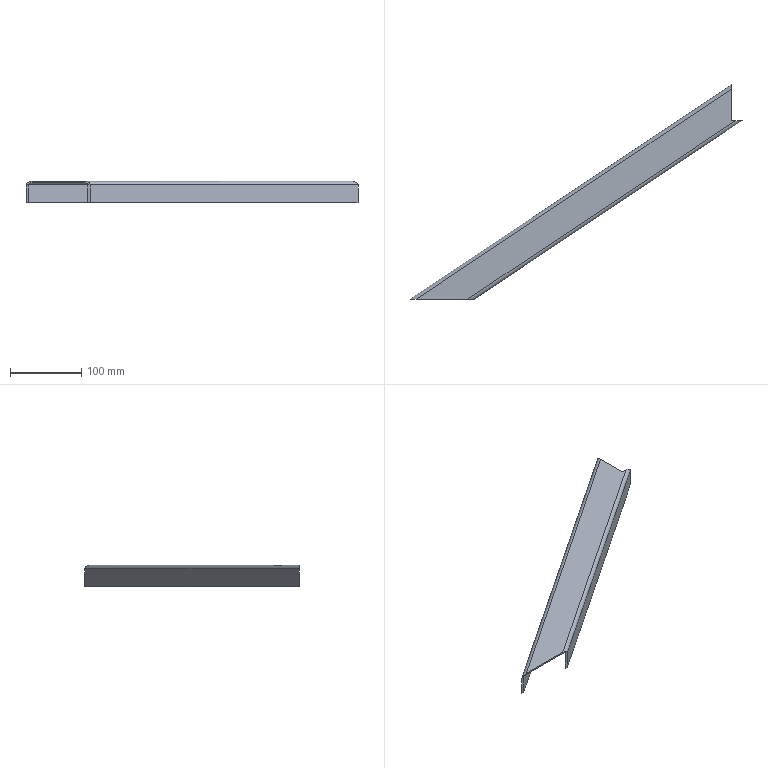Component | SolidWorks | 50x30x2ColdBentEqualAngleSteel500mm-1 | 1 solid | 15 faces | box 465.14 x 300 x 30 mm | volume 100821 mm3 | plane 11 | cylinder 4 | commonest cylinder face diameters 10 x2 6 x2
build123d program:
from build123d import *

# Parameters (mm, degrees)
BOSS_EXTRUDE1_DEPTH = 550
CUT_EXTRUDE4_DEPTH  = 88
CUT_EXTRUDE8_DEPTH  = 106


with BuildPart() as part:
    # Sketch1 → Boss-Extrude1 (new body)
    with BuildSketch(Plane(origin=(0, 0, 0), x_dir=(0, 0, -1), z_dir=(1, 0, 0))):
        with BuildLine():
            Line((0, 5), (0, 45))
            ThreePointArc((0, 45), (1.464, 48.536), (5, 50))
            Line((5, 50), (30, 50))
            Line((30, 50), (30, 48))
            Line((30, 48), (5, 48))
            ThreePointArc((5, 48), (2.879, 47.121), (2, 45))
            Line((2, 45), (2, 5))
            ThreePointArc((2, 5), (2.879, 2.879), (5, 2))
            Line((5, 2), (30, 2))
            Line((30, 2), (30, 0))
            Line((30, 0), (5, 0))
            ThreePointArc((5, 0), (1.464, 1.464), (0, 5))
        make_face()
    extrude(amount=BOSS_EXTRUDE1_DEPTH)

    # Sketch3 → Cut-Extrude4 (cut)
    with BuildSketch(Plane.XY):
        Polygon((550, 50), (522.265, 8.397), (548.518, -9.104), (550, 0), align=None)
    extrude(amount=-CUT_EXTRUDE4_DEPTH, mode=Mode.SUBTRACT)

    # Sketch7 → Cut-Extrude8 (cut)
    with BuildSketch(Plane.XY):
        Polygon((84.167, 0), (9.167, 50), (0, 50), (0, 36.249), (0, 0), align=None)
    extrude(amount=-CUT_EXTRUDE8_DEPTH, mode=Mode.SUBTRACT)


solid = part.part

# Placed as in the assembly
solid = solid.moved(Location((-604.263, -294.588, 415), (0, 0, 33.69)))
STEP:
#1=CARTESIAN_POINT('',(-6.865,2.051,16.142));
#2=VERTEX_POINT('',#1);
#3=CARTESIAN_POINT('',(-24.582,-9.76,16.142));
#4=VERTEX_POINT('',#3);
#5=CARTESIAN_POINT('',(-6.865,2.051,16.142));
#6=DIRECTION('',(-0.8321,-0.5547,-0.));
#7=VECTOR('',#6,39.37);
#8=LINE('',#5,#7);
#9=EDGE_CURVE('',#2,#4,#8,.T.);
#10=ORIENTED_EDGE('',*,*,#9,.T.);
#11=CARTESIAN_POINT('',(-24.227,-9.76,16.339));
#12=VERTEX_POINT('',#11);
#13=CARTESIAN_POINT('',(-24.582,-9.76,16.142));
#14=CARTESIAN_POINT('',(-24.582,-9.76,16.257));
#15=CARTESIAN_POINT('',(-24.435,-9.76,16.339));
#16=CARTESIAN_POINT('',(-24.227,-9.76,16.339));
#17=(BOUNDED_CURVE()B_SPLINE_CURVE(3,(#13,#14,#15,#16),.UNSPECIFIED.,.F.,.F.)B_SPLINE_CURVE_WITH_KNOTS((4,4),(-0.,1.571),.UNSPECIFIED.)CURVE()GEOMETRIC_REPRESENTATION_ITEM()RATIONAL_B_SPLINE_CURVE((1.,0.8047,0.8047,1.))REPRESENTATION_ITEM(''));
#18=EDGE_CURVE('',#4,#12,#17,.T.);
#19=ORIENTED_EDGE('',*,*,#18,.T.);
#20=CARTESIAN_POINT('',(-6.865,1.815,16.339));
#21=VERTEX_POINT('',#20);
#22=CARTESIAN_POINT('',(-6.756,1.887,16.339));
#23=DIRECTION('',(-0.8321,-0.5547,-0.));
#24=VECTOR('',#23,39.37);
#25=LINE('',#22,#24);
#26=EDGE_CURVE('',#21,#12,#25,.T.);
#27=ORIENTED_EDGE('',*,*,#26,.F.);
#28=CARTESIAN_POINT('',(-6.865,1.815,16.339));
#29=CARTESIAN_POINT('',(-6.865,1.953,16.339));
#30=CARTESIAN_POINT('',(-6.865,2.051,16.257));
#31=CARTESIAN_POINT('',(-6.865,2.051,16.142));
#32=(BOUNDED_CURVE()B_SPLINE_CURVE(3,(#28,#29,#30,#31),.UNSPECIFIED.,.F.,.F.)B_SPLINE_CURVE_WITH_KNOTS((4,4),(1.571,3.142),.UNSPECIFIED.)CURVE()GEOMETRIC_REPRESENTATION_ITEM()RATIONAL_B_SPLINE_CURVE((1.,0.8047,0.8047,1.))REPRESENTATION_ITEM(''));
#33=EDGE_CURVE('',#21,#2,#32,.T.);
#34=ORIENTED_EDGE('',*,*,#33,.T.);
#35=EDGE_LOOP('',(#10,#19,#27,#34));
#36=FACE_OUTER_BOUND('',#35,.T.);
#37=CARTESIAN_POINT('',(-6.756,1.887,16.142));
#38=DIRECTION('',(-0.8321,-0.5547,-0.));
#39=DIRECTION('',(0.,0.,1.));
#40=AXIS2_PLACEMENT_3D('',#37,#38,#39);
#41=CYLINDRICAL_SURFACE('',#40,0.1969);
#42=ADVANCED_FACE('',(#36),#41,.T.);
#43=ORIENTED_EDGE('',*,*,#26,.T.);
#44=CARTESIAN_POINT('',(-21.388,-9.76,16.339));
#45=VERTEX_POINT('',#44);
#46=CARTESIAN_POINT('',(-21.033,-9.76,16.339));
#47=DIRECTION('',(-1.,-0.,-0.));
#48=VECTOR('',#47,39.37);
#49=LINE('',#46,#48);
#50=EDGE_CURVE('',#45,#12,#49,.T.);
#51=ORIENTED_EDGE('',*,*,#50,.F.);
#52=CARTESIAN_POINT('',(-6.624,0.08267,16.339));
#53=VERTEX_POINT('',#52);
#54=CARTESIAN_POINT('',(-5.882,0.5771,16.339));
#55=DIRECTION('',(-0.8321,-0.5547,-0.));
#56=VECTOR('',#55,39.37);
#57=LINE('',#54,#56);
#58=EDGE_CURVE('',#53,#45,#57,.T.);
#59=ORIENTED_EDGE('',*,*,#58,.F.);
#60=CARTESIAN_POINT('',(-6.865,0.08267,16.339));
#61=VERTEX_POINT('',#60);
#62=CARTESIAN_POINT('',(-6.865,0.08267,16.339));
#63=DIRECTION('',(1.,0.,0.));
#64=VECTOR('',#63,39.37);
#65=LINE('',#62,#64);
#66=EDGE_CURVE('',#61,#53,#65,.T.);
#67=ORIENTED_EDGE('',*,*,#66,.F.);
#68=CARTESIAN_POINT('',(-6.865,2.051,16.339));
#69=DIRECTION('',(-0.,-1.,-0.));
#70=VECTOR('',#69,39.37);
#71=LINE('',#68,#70);
#72=EDGE_CURVE('',#21,#61,#71,.T.);
#73=ORIENTED_EDGE('',*,*,#72,.F.);
#74=EDGE_LOOP('',(#43,#51,#59,#67,#73));
#75=FACE_OUTER_BOUND('',#74,.T.);
#76=CARTESIAN_POINT('',(-5.882,0.5771,16.339));
#77=DIRECTION('',(0.,0.,-1.));
#78=DIRECTION('',(-0.8321,-0.5547,-0.));
#79=AXIS2_PLACEMENT_3D('',#76,#77,#78);
#80=PLANE('',#79);
#81=ADVANCED_FACE('',(#75),#80,.F.);
#82=ORIENTED_EDGE('',*,*,#58,.T.);
#83=CARTESIAN_POINT('',(-21.033,-9.76,16.142));
#84=VERTEX_POINT('',#83);
#85=CARTESIAN_POINT('',(-21.388,-9.76,16.339));
#86=CARTESIAN_POINT('',(-21.18,-9.76,16.339));
#87=CARTESIAN_POINT('',(-21.033,-9.76,16.257));
#88=CARTESIAN_POINT('',(-21.033,-9.76,16.142));
#89=(BOUNDED_CURVE()B_SPLINE_CURVE(3,(#85,#86,#87,#88),.UNSPECIFIED.,.F.,.F.)B_SPLINE_CURVE_WITH_KNOTS((4,4),(1.571,3.142),.UNSPECIFIED.)CURVE()GEOMETRIC_REPRESENTATION_ITEM()RATIONAL_B_SPLINE_CURVE((1.,0.8047,0.8047,1.))REPRESENTATION_ITEM(''));
#90=EDGE_CURVE('',#45,#84,#89,.T.);
#91=ORIENTED_EDGE('',*,*,#90,.T.);
#92=CARTESIAN_POINT('',(-6.269,0.08267,16.142));
#93=VERTEX_POINT('',#92);
#94=CARTESIAN_POINT('',(-5.773,0.4133,16.142));
#95=DIRECTION('',(-0.8321,-0.5547,-0.));
#96=VECTOR('',#95,39.37);
#97=LINE('',#94,#96);
#98=EDGE_CURVE('',#93,#84,#97,.T.);
#99=ORIENTED_EDGE('',*,*,#98,.F.);
#100=CARTESIAN_POINT('',(-6.269,0.08267,16.142));
#101=CARTESIAN_POINT('',(-6.269,0.08267,16.257));
#102=CARTESIAN_POINT('',(-6.416,0.08267,16.339));
#103=CARTESIAN_POINT('',(-6.624,0.08267,16.339));
#104=(BOUNDED_CURVE()B_SPLINE_CURVE(3,(#100,#101,#102,#103),.UNSPECIFIED.,.F.,.F.)B_SPLINE_CURVE_WITH_KNOTS((4,4),(3.142,4.712),.UNSPECIFIED.)CURVE()GEOMETRIC_REPRESENTATION_ITEM()RATIONAL_B_SPLINE_CURVE((1.,0.8047,0.8047,1.))REPRESENTATION_ITEM(''));
#105=EDGE_CURVE('',#93,#53,#104,.T.);
#106=ORIENTED_EDGE('',*,*,#105,.T.);
#107=EDGE_LOOP('',(#82,#91,#99,#106));
#108=FACE_OUTER_BOUND('',#107,.T.);
#109=CARTESIAN_POINT('',(-5.882,0.5771,16.142));
#110=DIRECTION('',(-0.8321,-0.5547,-0.));
#111=DIRECTION('',(0.,0.,1.));
#112=AXIS2_PLACEMENT_3D('',#109,#110,#111);
#113=CYLINDRICAL_SURFACE('',#112,0.1969);
#114=ADVANCED_FACE('',(#108),#113,.T.);
#115=ORIENTED_EDGE('',*,*,#98,.T.);
#116=CARTESIAN_POINT('',(-21.033,-9.76,15.157));
#117=VERTEX_POINT('',#116);
#118=CARTESIAN_POINT('',(-21.033,-9.76,12.165));
#119=DIRECTION('',(-0.,-0.,1.));
#120=VECTOR('',#119,39.37);
#121=LINE('',#118,#120);
#122=EDGE_CURVE('',#117,#84,#121,.T.);
#123=ORIENTED_EDGE('',*,*,#122,.F.);
#124=CARTESIAN_POINT('',(-6.269,0.08267,15.157));
#125=VERTEX_POINT('',#124);
#126=CARTESIAN_POINT('',(-5.773,0.4133,15.157));
#127=DIRECTION('',(-0.8321,-0.5547,-0.));
#128=VECTOR('',#127,39.37);
#129=LINE('',#126,#128);
#130=EDGE_CURVE('',#125,#117,#129,.T.);
#131=ORIENTED_EDGE('',*,*,#130,.F.);
#132=CARTESIAN_POINT('',(-6.269,0.08267,16.142));
#133=DIRECTION('',(-0.,-0.,1.));
#134=VECTOR('',#133,39.37);
#135=LINE('',#132,#134);
#136=EDGE_CURVE('',#125,#93,#135,.T.);
#137=ORIENTED_EDGE('',*,*,#136,.T.);
#138=EDGE_LOOP('',(#115,#123,#131,#137));
#139=FACE_OUTER_BOUND('',#138,.T.);
#140=CARTESIAN_POINT('',(-5.773,0.4133,16.142));
#141=DIRECTION('',(-0.5547,0.8321,-0.));
#142=DIRECTION('',(-0.,-0.,1.));
#143=AXIS2_PLACEMENT_3D('',#140,#141,#142);
#144=PLANE('',#143);
#145=ADVANCED_FACE('',(#139),#144,.F.);
#146=ORIENTED_EDGE('',*,*,#130,.T.);
#147=CARTESIAN_POINT('',(-21.175,-9.76,15.157));
#148=VERTEX_POINT('',#147);
#149=CARTESIAN_POINT('',(-5.817,-9.76,15.157));
#150=DIRECTION('',(-1.,-0.,-0.));
#151=VECTOR('',#150,39.37);
#152=LINE('',#149,#151);
#153=EDGE_CURVE('',#117,#148,#152,.T.);
#154=ORIENTED_EDGE('',*,*,#153,.T.);
#155=CARTESIAN_POINT('',(-6.411,0.08267,15.157));
#156=VERTEX_POINT('',#155);
#157=CARTESIAN_POINT('',(-5.817,0.4788,15.157));
#158=DIRECTION('',(-0.8321,-0.5547,-0.));
#159=VECTOR('',#158,39.37);
#160=LINE('',#157,#159);
#161=EDGE_CURVE('',#156,#148,#160,.T.);
#162=ORIENTED_EDGE('',*,*,#161,.F.);
#163=CARTESIAN_POINT('',(-5.817,0.08267,15.157));
#164=DIRECTION('',(1.,0.,0.));
#165=VECTOR('',#164,39.37);
#166=LINE('',#163,#165);
#167=EDGE_CURVE('',#156,#125,#166,.T.);
#168=ORIENTED_EDGE('',*,*,#167,.T.);
#169=EDGE_LOOP('',(#146,#154,#162,#168));
#170=FACE_OUTER_BOUND('',#169,.T.);
#171=CARTESIAN_POINT('',(-5.817,0.4788,15.157));
#172=DIRECTION('',(-0.,-0.,1.));
#173=DIRECTION('',(0.8321,0.5547,0.));
#174=AXIS2_PLACEMENT_3D('',#171,#172,#173);
#175=PLANE('',#174);
#176=ADVANCED_FACE('',(#170),#175,.F.);
#177=ORIENTED_EDGE('',*,*,#161,.T.);
#178=CARTESIAN_POINT('',(-21.175,-9.76,16.142));
#179=VERTEX_POINT('',#178);
#180=CARTESIAN_POINT('',(-21.175,-9.76,16.142));
#181=DIRECTION('',(-0.,-0.,1.));
#182=VECTOR('',#181,39.37);
#183=LINE('',#180,#182);
#184=EDGE_CURVE('',#148,#179,#183,.T.);
#185=ORIENTED_EDGE('',*,*,#184,.T.);
#186=CARTESIAN_POINT('',(-6.411,0.08267,16.142));
#187=VERTEX_POINT('',#186);
#188=CARTESIAN_POINT('',(-5.817,0.4788,16.142));
#189=DIRECTION('',(-0.8321,-0.5547,-0.));
#190=VECTOR('',#189,39.37);
#191=LINE('',#188,#190);
#192=EDGE_CURVE('',#187,#179,#191,.T.);
#193=ORIENTED_EDGE('',*,*,#192,.F.);
#194=CARTESIAN_POINT('',(-6.411,0.08267,16.142));
#195=DIRECTION('',(0.,0.,-1.));
#196=VECTOR('',#195,39.37);
#197=LINE('',#194,#196);
#198=EDGE_CURVE('',#187,#156,#197,.T.);
#199=ORIENTED_EDGE('',*,*,#198,.T.);
#200=EDGE_LOOP('',(#177,#185,#193,#199));
#201=FACE_OUTER_BOUND('',#200,.T.);
#202=CARTESIAN_POINT('',(-5.817,0.4788,16.142));
#203=DIRECTION('',(0.5547,-0.8321,0.));
#204=DIRECTION('',(0.,0.,-1.));
#205=AXIS2_PLACEMENT_3D('',#202,#203,#204);
#206=PLANE('',#205);
#207=ADVANCED_FACE('',(#201),#206,.F.);
#208=ORIENTED_EDGE('',*,*,#192,.T.);
#209=CARTESIAN_POINT('',(-21.388,-9.76,16.26));
#210=VERTEX_POINT('',#209);
#211=CARTESIAN_POINT('',(-21.175,-9.76,16.142));
#212=CARTESIAN_POINT('',(-21.175,-9.76,16.211));
#213=CARTESIAN_POINT('',(-21.263,-9.76,16.26));
#214=CARTESIAN_POINT('',(-21.388,-9.76,16.26));
#215=(BOUNDED_CURVE()B_SPLINE_CURVE(3,(#211,#212,#213,#214),.UNSPECIFIED.,.F.,.F.)B_SPLINE_CURVE_WITH_KNOTS((4,4),(3.142,4.712),.UNSPECIFIED.)CURVE()GEOMETRIC_REPRESENTATION_ITEM()RATIONAL_B_SPLINE_CURVE((1.,0.8047,0.8047,1.))REPRESENTATION_ITEM(''));
#216=EDGE_CURVE('',#179,#210,#215,.T.);
#217=ORIENTED_EDGE('',*,*,#216,.T.);
#218=CARTESIAN_POINT('',(-6.624,0.08267,16.26));
#219=VERTEX_POINT('',#218);
#220=CARTESIAN_POINT('',(-5.882,0.5771,16.26));
#221=DIRECTION('',(-0.8321,-0.5547,-0.));
#222=VECTOR('',#221,39.37);
#223=LINE('',#220,#222);
#224=EDGE_CURVE('',#219,#210,#223,.T.);
#225=ORIENTED_EDGE('',*,*,#224,.F.);
#226=CARTESIAN_POINT('',(-6.624,0.08267,16.26));
#227=CARTESIAN_POINT('',(-6.499,0.08267,16.26));
#228=CARTESIAN_POINT('',(-6.411,0.08267,16.211));
#229=CARTESIAN_POINT('',(-6.411,0.08267,16.142));
#230=(BOUNDED_CURVE()B_SPLINE_CURVE(3,(#226,#227,#228,#229),.UNSPECIFIED.,.F.,.F.)B_SPLINE_CURVE_WITH_KNOTS((4,4),(1.571,3.142),.UNSPECIFIED.)CURVE()GEOMETRIC_REPRESENTATION_ITEM()RATIONAL_B_SPLINE_CURVE((1.,0.8047,0.8047,1.))REPRESENTATION_ITEM(''));
#231=EDGE_CURVE('',#219,#187,#230,.T.);
#232=ORIENTED_EDGE('',*,*,#231,.T.);
#233=EDGE_LOOP('',(#208,#217,#225,#232));
#234=FACE_OUTER_BOUND('',#233,.T.);
#235=CARTESIAN_POINT('',(-5.882,0.5771,16.142));
#236=DIRECTION('',(-0.8321,-0.5547,-0.));
#237=DIRECTION('',(0.,0.,1.));
#238=AXIS2_PLACEMENT_3D('',#235,#236,#237);
#239=CYLINDRICAL_SURFACE('',#238,0.1181);
#240=ADVANCED_FACE('',(#234),#239,.F.);
#241=ORIENTED_EDGE('',*,*,#224,.T.);
#242=CARTESIAN_POINT('',(-24.227,-9.76,16.26));
#243=VERTEX_POINT('',#242);
#244=CARTESIAN_POINT('',(-5.882,-9.76,16.26));
#245=DIRECTION('',(-1.,-0.,-0.));
#246=VECTOR('',#245,39.37);
#247=LINE('',#244,#246);
#248=EDGE_CURVE('',#210,#243,#247,.T.);
#249=ORIENTED_EDGE('',*,*,#248,.T.);
#250=CARTESIAN_POINT('',(-6.865,1.815,16.26));
#251=VERTEX_POINT('',#250);
#252=CARTESIAN_POINT('',(-6.756,1.887,16.26));
#253=DIRECTION('',(-0.8321,-0.5547,-0.));
#254=VECTOR('',#253,39.37);
#255=LINE('',#252,#254);
#256=EDGE_CURVE('',#251,#243,#255,.T.);
#257=ORIENTED_EDGE('',*,*,#256,.F.);
#258=CARTESIAN_POINT('',(-6.865,0.08267,16.26));
#259=VERTEX_POINT('',#258);
#260=CARTESIAN_POINT('',(-6.865,0.5771,16.26));
#261=DIRECTION('',(-0.,-1.,-0.));
#262=VECTOR('',#261,39.37);
#263=LINE('',#260,#262);
#264=EDGE_CURVE('',#251,#259,#263,.T.);
#265=ORIENTED_EDGE('',*,*,#264,.T.);
#266=CARTESIAN_POINT('',(-5.882,0.08267,16.26));
#267=DIRECTION('',(1.,0.,0.));
#268=VECTOR('',#267,39.37);
#269=LINE('',#266,#268);
#270=EDGE_CURVE('',#259,#219,#269,.T.);
#271=ORIENTED_EDGE('',*,*,#270,.T.);
#272=EDGE_LOOP('',(#241,#249,#257,#265,#271));
#273=FACE_OUTER_BOUND('',#272,.T.);
#274=CARTESIAN_POINT('',(-5.882,0.5771,16.26));
#275=DIRECTION('',(-0.,-0.,1.));
#276=DIRECTION('',(0.8321,0.5547,0.));
#277=AXIS2_PLACEMENT_3D('',#274,#275,#276);
#278=PLANE('',#277);
#279=ADVANCED_FACE('',(#273),#278,.F.);
#280=ORIENTED_EDGE('',*,*,#256,.T.);
#281=CARTESIAN_POINT('',(-24.44,-9.76,16.142));
#282=VERTEX_POINT('',#281);
#283=CARTESIAN_POINT('',(-24.227,-9.76,16.26));
#284=CARTESIAN_POINT('',(-24.351,-9.76,16.26));
#285=CARTESIAN_POINT('',(-24.44,-9.76,16.211));
#286=CARTESIAN_POINT('',(-24.44,-9.76,16.142));
#287=(BOUNDED_CURVE()B_SPLINE_CURVE(3,(#283,#284,#285,#286),.UNSPECIFIED.,.F.,.F.)B_SPLINE_CURVE_WITH_KNOTS((4,4),(4.712,6.283),.UNSPECIFIED.)CURVE()GEOMETRIC_REPRESENTATION_ITEM()RATIONAL_B_SPLINE_CURVE((1.,0.8047,0.8047,1.))REPRESENTATION_ITEM(''));
#288=EDGE_CURVE('',#243,#282,#287,.T.);
#289=ORIENTED_EDGE('',*,*,#288,.T.);
#290=CARTESIAN_POINT('',(-6.865,1.957,16.142));
#291=VERTEX_POINT('',#290);
#292=CARTESIAN_POINT('',(-6.821,1.986,16.142));
#293=DIRECTION('',(-0.8321,-0.5547,-0.));
#294=VECTOR('',#293,39.37);
#295=LINE('',#292,#294);
#296=EDGE_CURVE('',#291,#282,#295,.T.);
#297=ORIENTED_EDGE('',*,*,#296,.F.);
#298=CARTESIAN_POINT('',(-6.865,1.957,16.142));
#299=CARTESIAN_POINT('',(-6.865,1.957,16.211));
#300=CARTESIAN_POINT('',(-6.865,1.898,16.26));
#301=CARTESIAN_POINT('',(-6.865,1.815,16.26));
#302=(BOUNDED_CURVE()B_SPLINE_CURVE(3,(#298,#299,#300,#301),.UNSPECIFIED.,.F.,.F.)B_SPLINE_CURVE_WITH_KNOTS((4,4),(3.142,4.712),.UNSPECIFIED.)CURVE()GEOMETRIC_REPRESENTATION_ITEM()RATIONAL_B_SPLINE_CURVE((1.,0.8047,0.8047,1.))REPRESENTATION_ITEM(''));
#303=EDGE_CURVE('',#291,#251,#302,.T.);
#304=ORIENTED_EDGE('',*,*,#303,.T.);
#305=EDGE_LOOP('',(#280,#289,#297,#304));
#306=FACE_OUTER_BOUND('',#305,.T.);
#307=CARTESIAN_POINT('',(-6.756,1.887,16.142));
#308=DIRECTION('',(-0.8321,-0.5547,-0.));
#309=DIRECTION('',(0.,0.,1.));
#310=AXIS2_PLACEMENT_3D('',#307,#308,#309);
#311=CYLINDRICAL_SURFACE('',#310,0.1181);
#312=ADVANCED_FACE('',(#306),#311,.F.);
#313=ORIENTED_EDGE('',*,*,#296,.T.);
#314=CARTESIAN_POINT('',(-24.44,-9.76,15.157));
#315=VERTEX_POINT('',#314);
#316=CARTESIAN_POINT('',(-24.44,-9.76,16.142));
#317=DIRECTION('',(0.,0.,-1.));
#318=VECTOR('',#317,39.37);
#319=LINE('',#316,#318);
#320=EDGE_CURVE('',#282,#315,#319,.T.);
#321=ORIENTED_EDGE('',*,*,#320,.T.);
#322=CARTESIAN_POINT('',(-6.865,1.957,15.157));
#323=VERTEX_POINT('',#322);
#324=CARTESIAN_POINT('',(-6.821,1.986,15.157));
#325=DIRECTION('',(-0.8321,-0.5547,-0.));
#326=VECTOR('',#325,39.37);
#327=LINE('',#324,#326);
#328=EDGE_CURVE('',#323,#315,#327,.T.);
#329=ORIENTED_EDGE('',*,*,#328,.F.);
#330=CARTESIAN_POINT('',(-6.865,1.957,16.142));
#331=DIRECTION('',(-0.,-0.,1.));
#332=VECTOR('',#331,39.37);
#333=LINE('',#330,#332);
#334=EDGE_CURVE('',#323,#291,#333,.T.);
#335=ORIENTED_EDGE('',*,*,#334,.T.);
#336=EDGE_LOOP('',(#313,#321,#329,#335));
#337=FACE_OUTER_BOUND('',#336,.T.);
#338=CARTESIAN_POINT('',(-6.821,1.986,16.142));
#339=DIRECTION('',(-0.5547,0.8321,-0.));
#340=DIRECTION('',(-0.,-0.,1.));
#341=AXIS2_PLACEMENT_3D('',#338,#339,#340);
#342=PLANE('',#341);
#343=ADVANCED_FACE('',(#337),#342,.F.);
#344=ORIENTED_EDGE('',*,*,#328,.T.);
#345=CARTESIAN_POINT('',(-24.582,-9.76,15.157));
#346=VERTEX_POINT('',#345);
#347=CARTESIAN_POINT('',(-6.865,-9.76,15.157));
#348=DIRECTION('',(-1.,-0.,-0.));
#349=VECTOR('',#348,39.37);
#350=LINE('',#347,#349);
#351=EDGE_CURVE('',#315,#346,#350,.T.);
#352=ORIENTED_EDGE('',*,*,#351,.T.);
#353=CARTESIAN_POINT('',(-6.865,2.051,15.157));
#354=VERTEX_POINT('',#353);
#355=CARTESIAN_POINT('',(-6.865,2.051,15.157));
#356=DIRECTION('',(-0.8321,-0.5547,-0.));
#357=VECTOR('',#356,39.37);
#358=LINE('',#355,#357);
#359=EDGE_CURVE('',#354,#346,#358,.T.);
#360=ORIENTED_EDGE('',*,*,#359,.F.);
#361=CARTESIAN_POINT('',(-6.865,2.051,15.157));
#362=DIRECTION('',(-0.,-1.,-0.));
#363=VECTOR('',#362,39.37);
#364=LINE('',#361,#363);
#365=EDGE_CURVE('',#354,#323,#364,.T.);
#366=ORIENTED_EDGE('',*,*,#365,.T.);
#367=EDGE_LOOP('',(#344,#352,#360,#366));
#368=FACE_OUTER_BOUND('',#367,.T.);
#369=CARTESIAN_POINT('',(-6.865,2.051,15.157));
#370=DIRECTION('',(-0.,-0.,1.));
#371=DIRECTION('',(0.8321,0.5547,0.));
#372=AXIS2_PLACEMENT_3D('',#369,#370,#371);
#373=PLANE('',#372);
#374=ADVANCED_FACE('',(#368),#373,.F.);
#375=ORIENTED_EDGE('',*,*,#359,.T.);
#376=CARTESIAN_POINT('',(-24.582,-9.76,12.165));
#377=DIRECTION('',(-0.,-0.,1.));
#378=VECTOR('',#377,39.37);
#379=LINE('',#376,#378);
#380=EDGE_CURVE('',#346,#4,#379,.T.);
#381=ORIENTED_EDGE('',*,*,#380,.T.);
#382=ORIENTED_EDGE('',*,*,#9,.F.);
#383=CARTESIAN_POINT('',(-6.865,2.051,16.142));
#384=DIRECTION('',(-0.,-0.,1.));
#385=VECTOR('',#384,39.37);
#386=LINE('',#383,#385);
#387=EDGE_CURVE('',#354,#2,#386,.T.);
#388=ORIENTED_EDGE('',*,*,#387,.F.);
#389=EDGE_LOOP('',(#375,#381,#382,#388));
#390=FACE_OUTER_BOUND('',#389,.T.);
#391=CARTESIAN_POINT('',(-6.865,2.051,16.142));
#392=DIRECTION('',(0.5547,-0.8321,0.));
#393=DIRECTION('',(0.,0.,-1.));
#394=AXIS2_PLACEMENT_3D('',#391,#392,#393);
#395=PLANE('',#394);
#396=ADVANCED_FACE('',(#390),#395,.F.);
#397=ORIENTED_EDGE('',*,*,#136,.F.);
#398=ORIENTED_EDGE('',*,*,#167,.F.);
#399=ORIENTED_EDGE('',*,*,#198,.F.);
#400=ORIENTED_EDGE('',*,*,#231,.F.);
#401=ORIENTED_EDGE('',*,*,#270,.F.);
#402=CARTESIAN_POINT('',(-6.865,0.08267,12.874));
#403=DIRECTION('',(-0.,-0.,1.));
#404=VECTOR('',#403,39.37);
#405=LINE('',#402,#404);
#406=EDGE_CURVE('',#259,#61,#405,.T.);
#407=ORIENTED_EDGE('',*,*,#406,.T.);
#408=ORIENTED_EDGE('',*,*,#66,.T.);
#409=ORIENTED_EDGE('',*,*,#105,.F.);
#410=EDGE_LOOP('',(#397,#398,#399,#400,#401,#407,#408,#409));
#411=FACE_OUTER_BOUND('',#410,.T.);
#412=CARTESIAN_POINT('',(-6.865,0.08267,12.874));
#413=DIRECTION('',(0.,-1.,-0.));
#414=DIRECTION('',(1.,0.,0.));
#415=AXIS2_PLACEMENT_3D('',#412,#413,#414);
#416=PLANE('',#415);
#417=ADVANCED_FACE('',(#411),#416,.F.);
#418=ORIENTED_EDGE('',*,*,#72,.T.);
#419=ORIENTED_EDGE('',*,*,#406,.F.);
#420=ORIENTED_EDGE('',*,*,#264,.F.);
#421=ORIENTED_EDGE('',*,*,#303,.F.);
#422=ORIENTED_EDGE('',*,*,#334,.F.);
#423=ORIENTED_EDGE('',*,*,#365,.F.);
#424=ORIENTED_EDGE('',*,*,#387,.T.);
#425=ORIENTED_EDGE('',*,*,#33,.F.);
#426=EDGE_LOOP('',(#418,#419,#420,#421,#422,#423,#424,#425));
#427=FACE_OUTER_BOUND('',#426,.T.);
#428=CARTESIAN_POINT('',(-6.865,2.051,12.874));
#429=DIRECTION('',(-1.,0.,-0.));
#430=DIRECTION('',(-0.,-1.,-0.));
#431=AXIS2_PLACEMENT_3D('',#428,#429,#430);
#432=PLANE('',#431);
#433=ADVANCED_FACE('',(#427),#432,.F.);
#434=ORIENTED_EDGE('',*,*,#380,.F.);
#435=ORIENTED_EDGE('',*,*,#351,.F.);
#436=ORIENTED_EDGE('',*,*,#320,.F.);
#437=ORIENTED_EDGE('',*,*,#288,.F.);
#438=ORIENTED_EDGE('',*,*,#248,.F.);
#439=ORIENTED_EDGE('',*,*,#216,.F.);
#440=ORIENTED_EDGE('',*,*,#184,.F.);
#441=ORIENTED_EDGE('',*,*,#153,.F.);
#442=ORIENTED_EDGE('',*,*,#122,.T.);
#443=ORIENTED_EDGE('',*,*,#90,.F.);
#444=ORIENTED_EDGE('',*,*,#50,.T.);
#445=ORIENTED_EDGE('',*,*,#18,.F.);
#446=EDGE_LOOP('',(#434,#435,#436,#437,#438,#439,#440,#441,#442,#443,#444,#445));
#447=FACE_OUTER_BOUND('',#446,.T.);
#448=CARTESIAN_POINT('',(-21.033,-9.76,12.165));
#449=DIRECTION('',(-0.,1.,0.));
#450=DIRECTION('',(-1.,-0.,-0.));
#451=AXIS2_PLACEMENT_3D('',#448,#449,#450);
#452=PLANE('',#451);
#453=ADVANCED_FACE('',(#447),#452,.F.);
#454=CLOSED_SHELL('',(#42,#81,#114,#145,#176,#207,#240,#279,#312,#343,#374,#396,#417,#433,#453));
#455=MANIFOLD_SOLID_BREP('',#454);
#456=CARTESIAN_POINT('',(0.,0.,0.));
#457=DIRECTION('',(0.,0.,1.));
#458=DIRECTION('',(1.,0.,0.));
#459=AXIS2_PLACEMENT_3D('',#456,#457,#458);
#460=(LENGTH_UNIT()NAMED_UNIT(*)SI_UNIT($,.METRE.));
#461=LENGTH_MEASURE_WITH_UNIT(LENGTH_MEASURE(0.0254),#460);
#462=DIMENSIONAL_EXPONENTS(1.,0.,0.,0.,0.,0.,0.);
#463=(CONVERSION_BASED_UNIT('',#461)LENGTH_UNIT()NAMED_UNIT(#462));
#464=UNCERTAINTY_MEASURE_WITH_UNIT(LENGTH_MEASURE(0.00001),#463,'','');
#465=(NAMED_UNIT(*)PLANE_ANGLE_UNIT()SI_UNIT($,.RADIAN.));
#466=(NAMED_UNIT(*)SI_UNIT($,.STERADIAN.)SOLID_ANGLE_UNIT());
#467=(GEOMETRIC_REPRESENTATION_CONTEXT(3)GLOBAL_UNCERTAINTY_ASSIGNED_CONTEXT((#464))GLOBAL_UNIT_ASSIGNED_CONTEXT((#463,#465,#466))REPRESENTATION_CONTEXT('',''));
#468=ADVANCED_BREP_SHAPE_REPRESENTATION('',(#455,#459),#467);
#469=COLOUR_RGB('',0.7922,0.8196,0.9333);
#470=FILL_AREA_STYLE_COLOUR('',#469);
#471=FILL_AREA_STYLE('',(#470));
#472=SURFACE_STYLE_FILL_AREA(#471);
#473=SURFACE_SIDE_STYLE('',(#472));
#474=SURFACE_STYLE_USAGE(.BOTH.,#473);
#475=PRESENTATION_STYLE_ASSIGNMENT((#474));
#476=STYLED_ITEM('',(#475),#455);
#477=PRESENTATION_LAYER_ASSIGNMENT('','',(#476));
#478=(LENGTH_UNIT()NAMED_UNIT(*)SI_UNIT($,.METRE.));
#479=LENGTH_MEASURE_WITH_UNIT(LENGTH_MEASURE(0.0254),#478);
#480=DIMENSIONAL_EXPONENTS(1.,0.,0.,0.,0.,0.,0.);
#481=(CONVERSION_BASED_UNIT('',#479)LENGTH_UNIT()NAMED_UNIT(#480));
#482=UNCERTAINTY_MEASURE_WITH_UNIT(LENGTH_MEASURE(0.00001),#481,'','');
#483=(NAMED_UNIT(*)PLANE_ANGLE_UNIT()SI_UNIT($,.RADIAN.));
#484=(NAMED_UNIT(*)SI_UNIT($,.STERADIAN.)SOLID_ANGLE_UNIT());
#485=(GEOMETRIC_REPRESENTATION_CONTEXT(3)GLOBAL_UNCERTAINTY_ASSIGNED_CONTEXT((#482))GLOBAL_UNIT_ASSIGNED_CONTEXT((#481,#483,#484))REPRESENTATION_CONTEXT('',''));
#486=MECHANICAL_DESIGN_GEOMETRIC_PRESENTATION_REPRESENTATION('',(#476),#485);